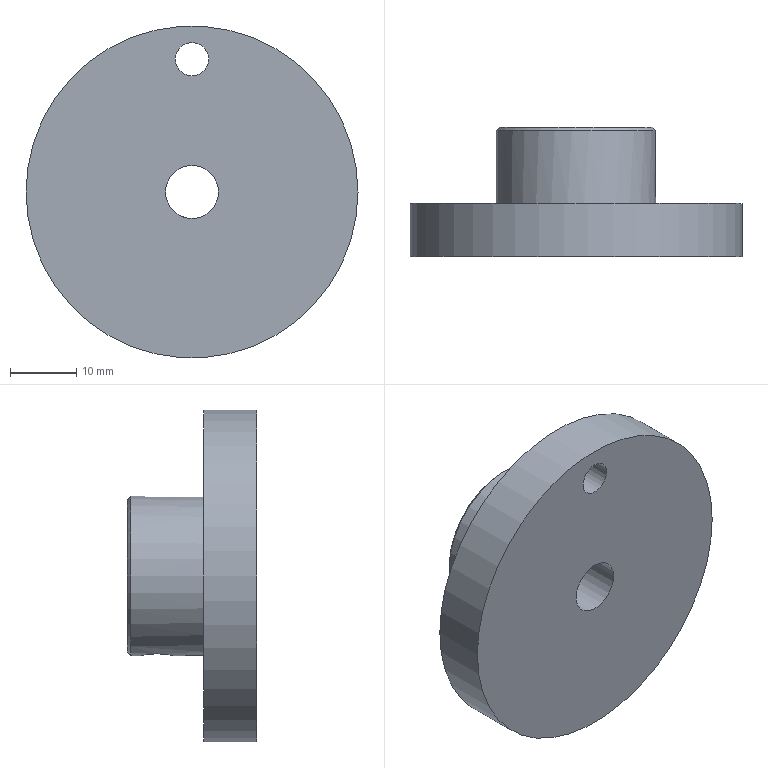Component | NX | HANDWHEEL | 1 solid | 9 faces | volume 19604 mm3 | cylinder 5 | plane 3 | cone 1 | commonest cylinder face diameters 5 x2 24 x1 8 x1 50 x1